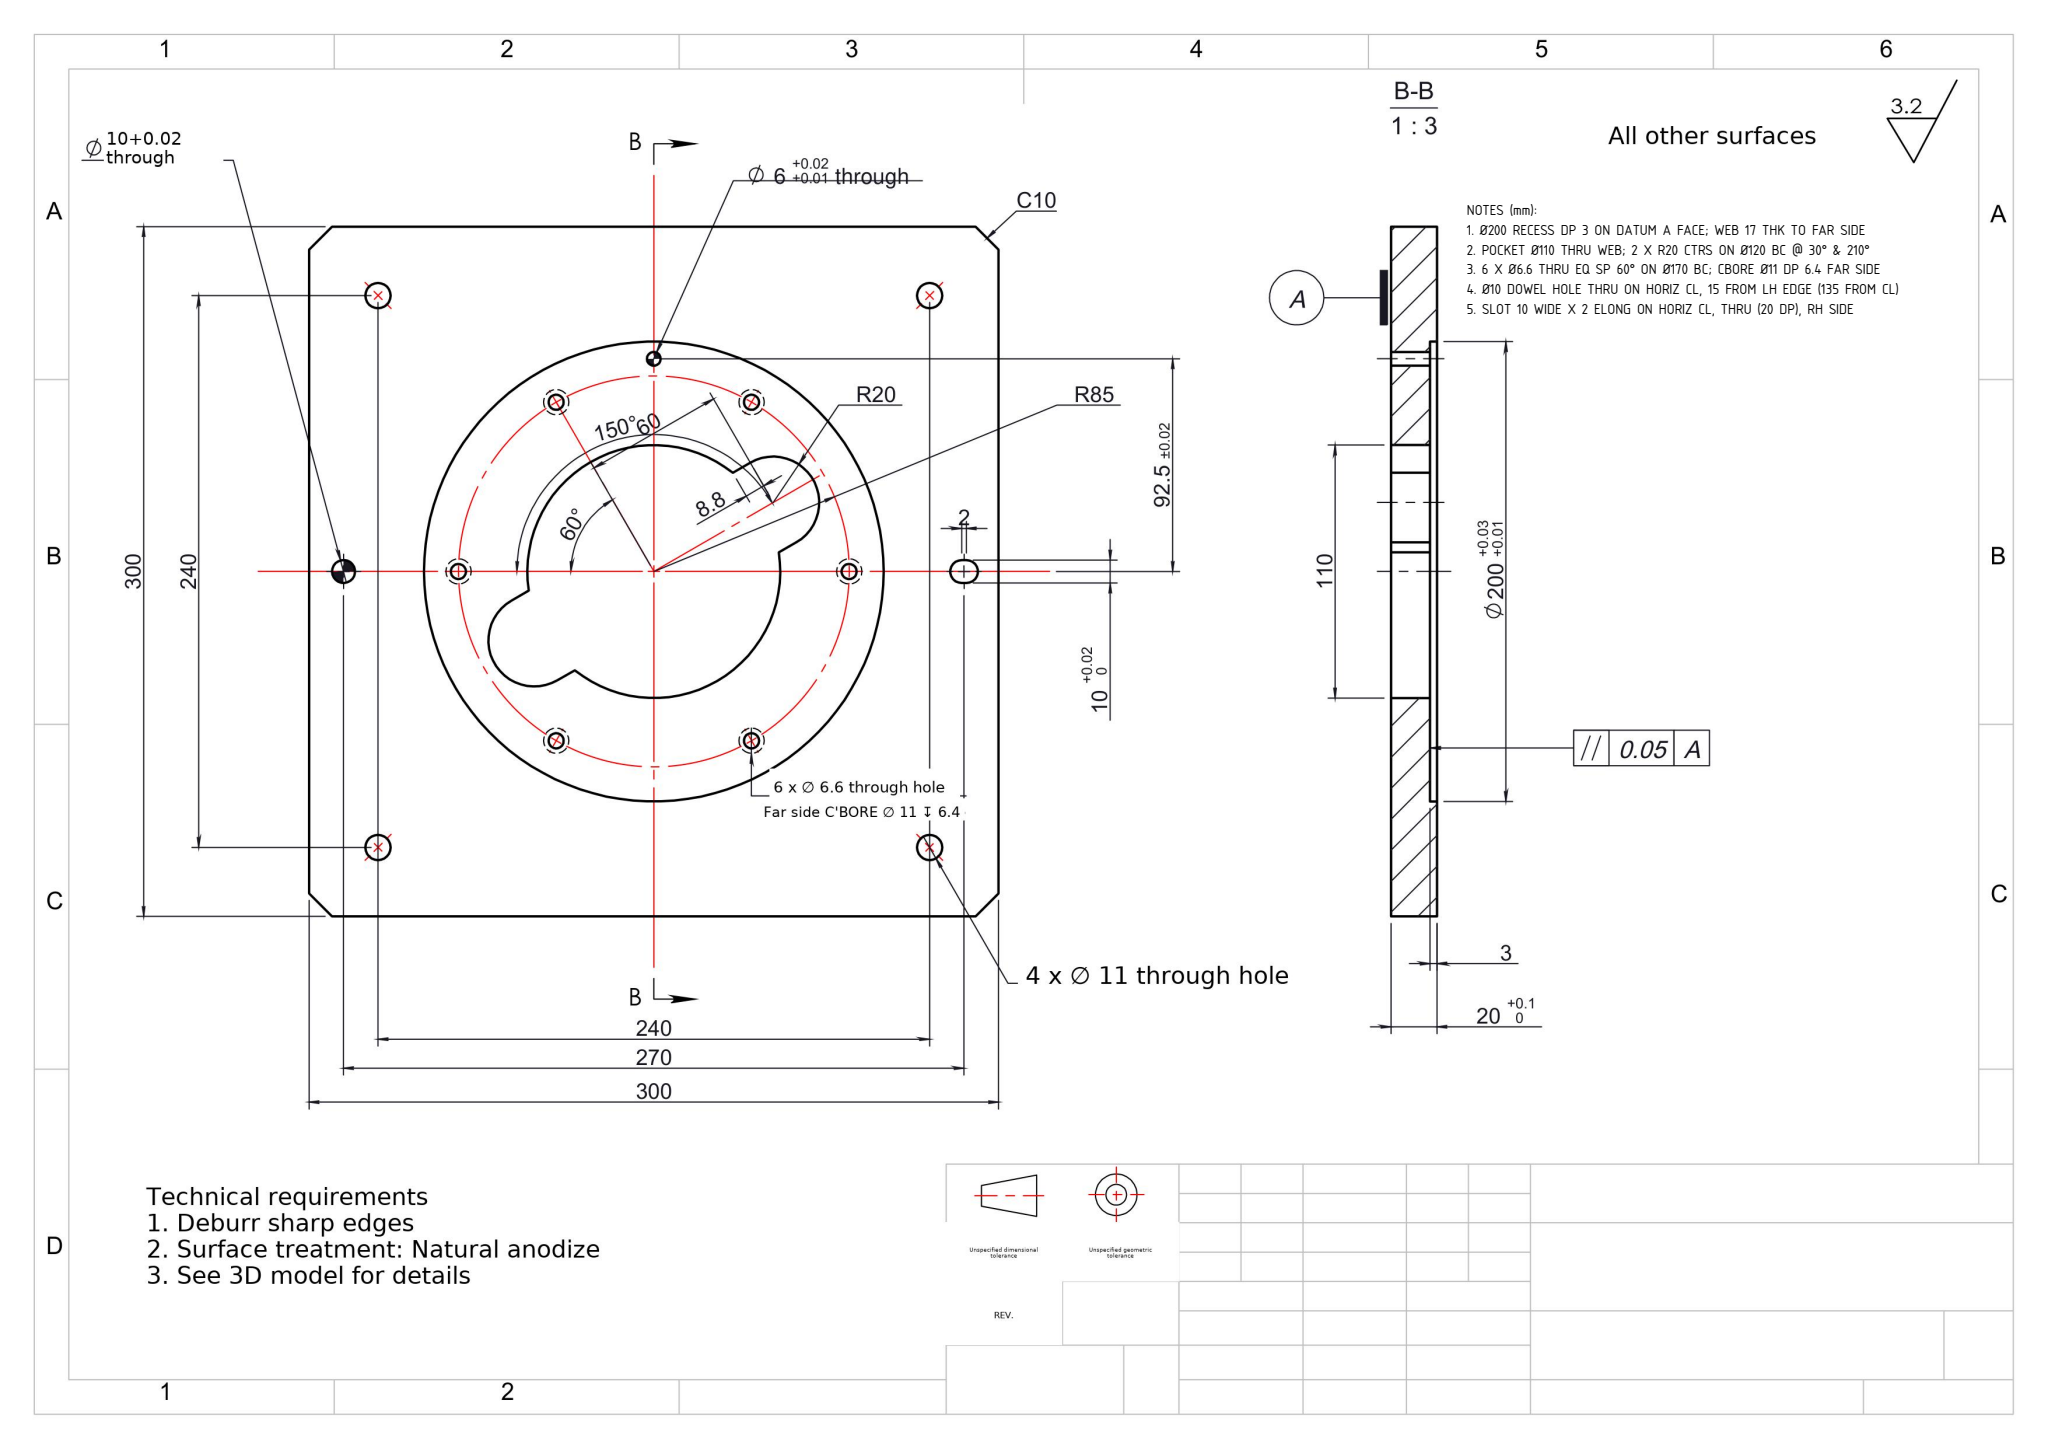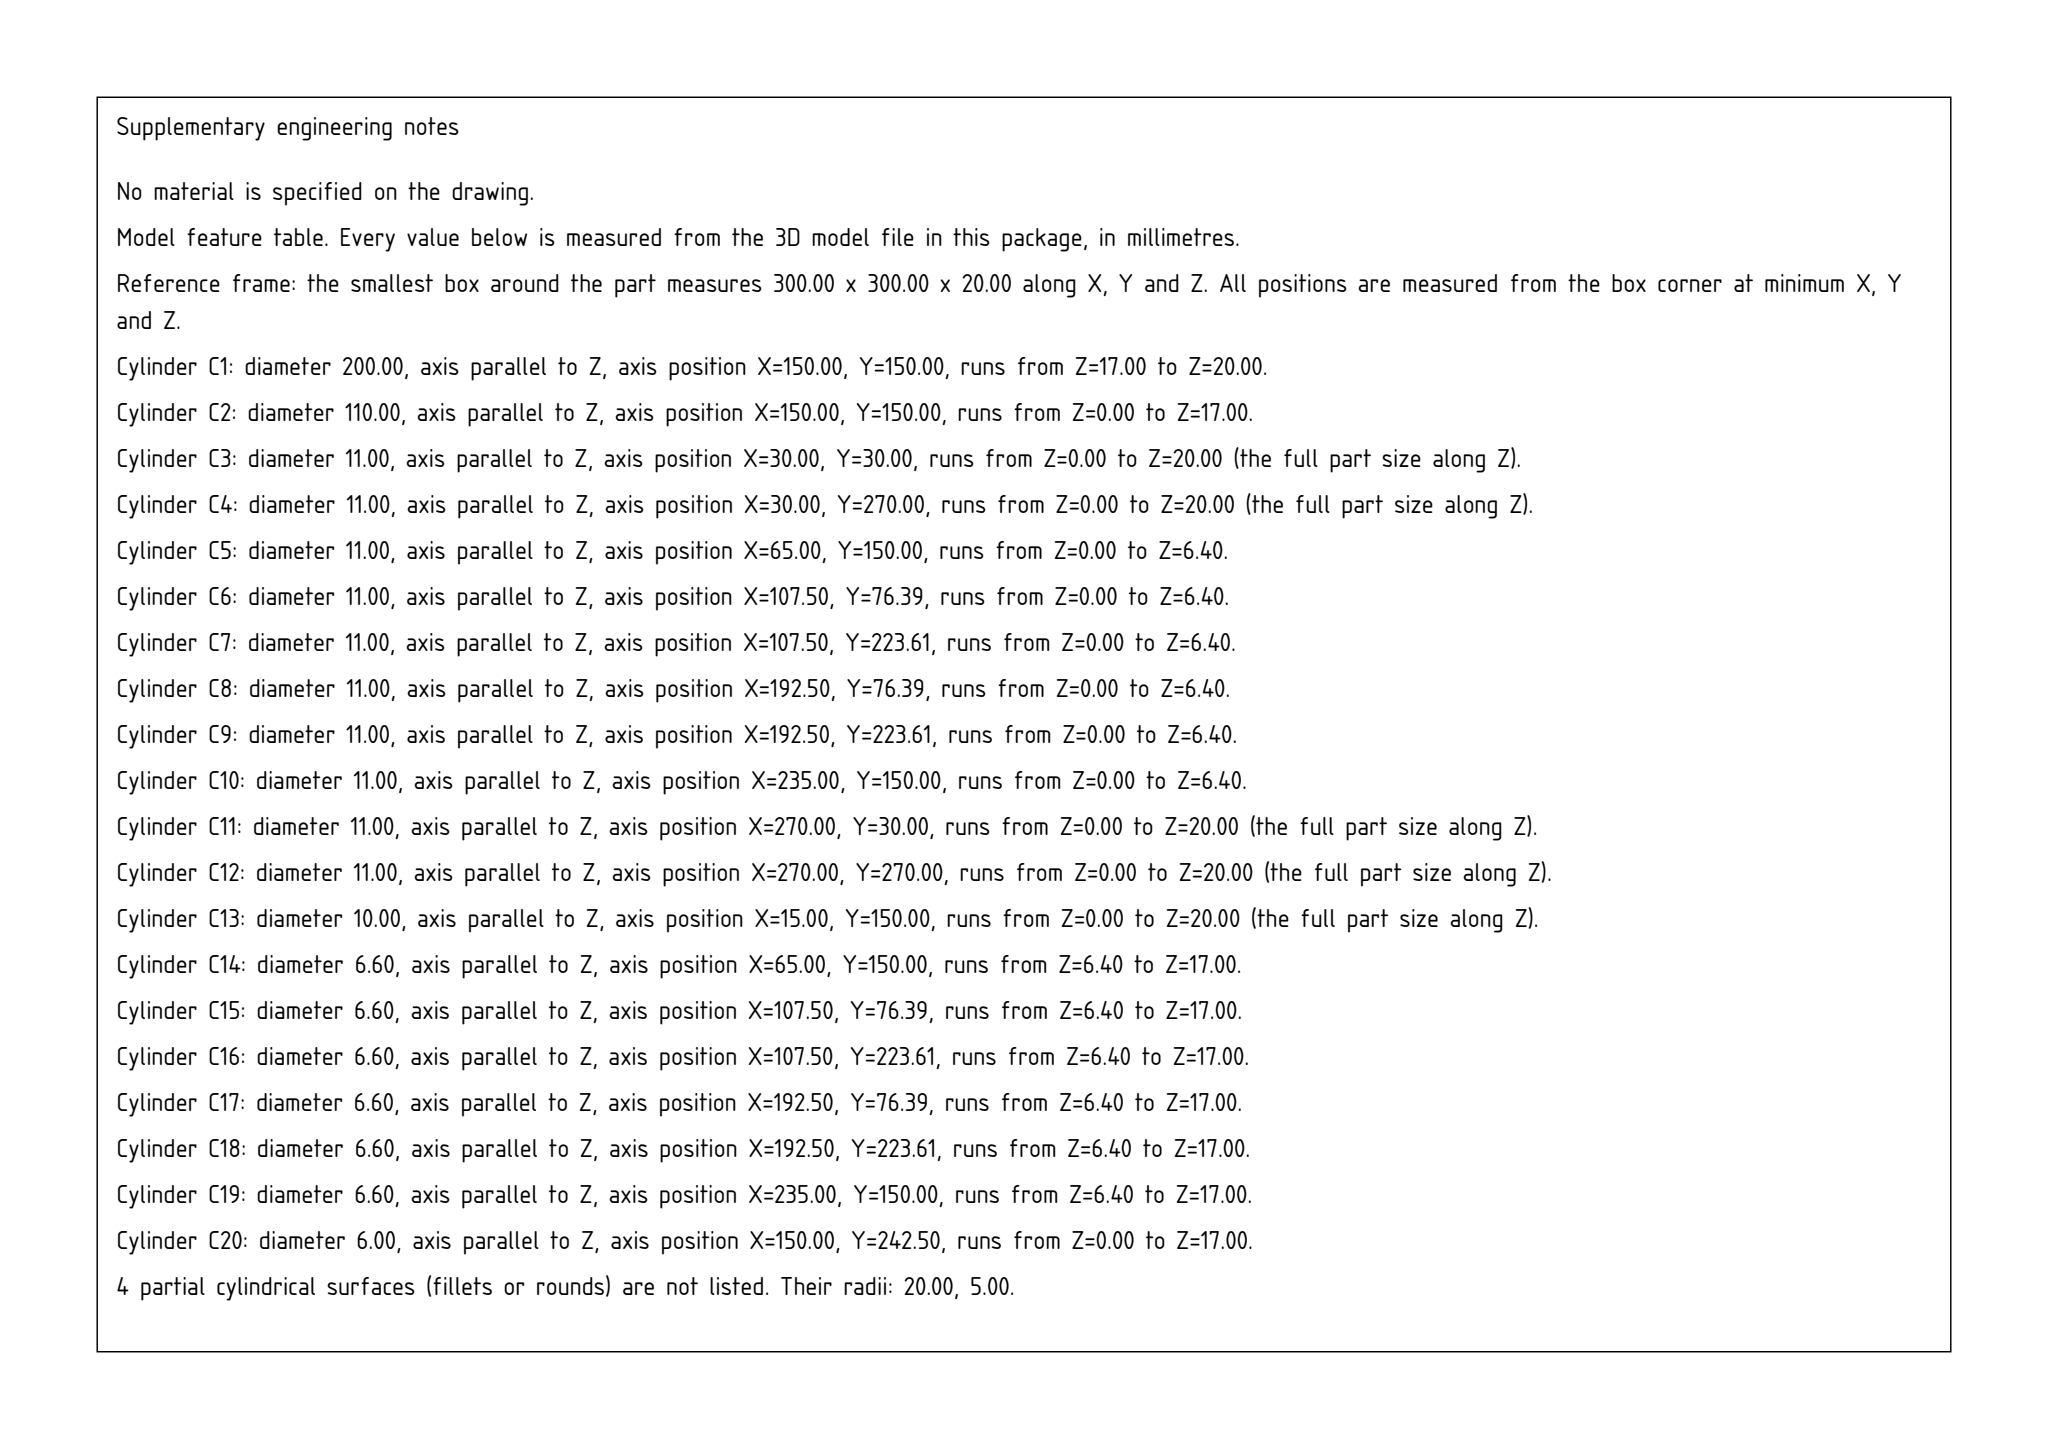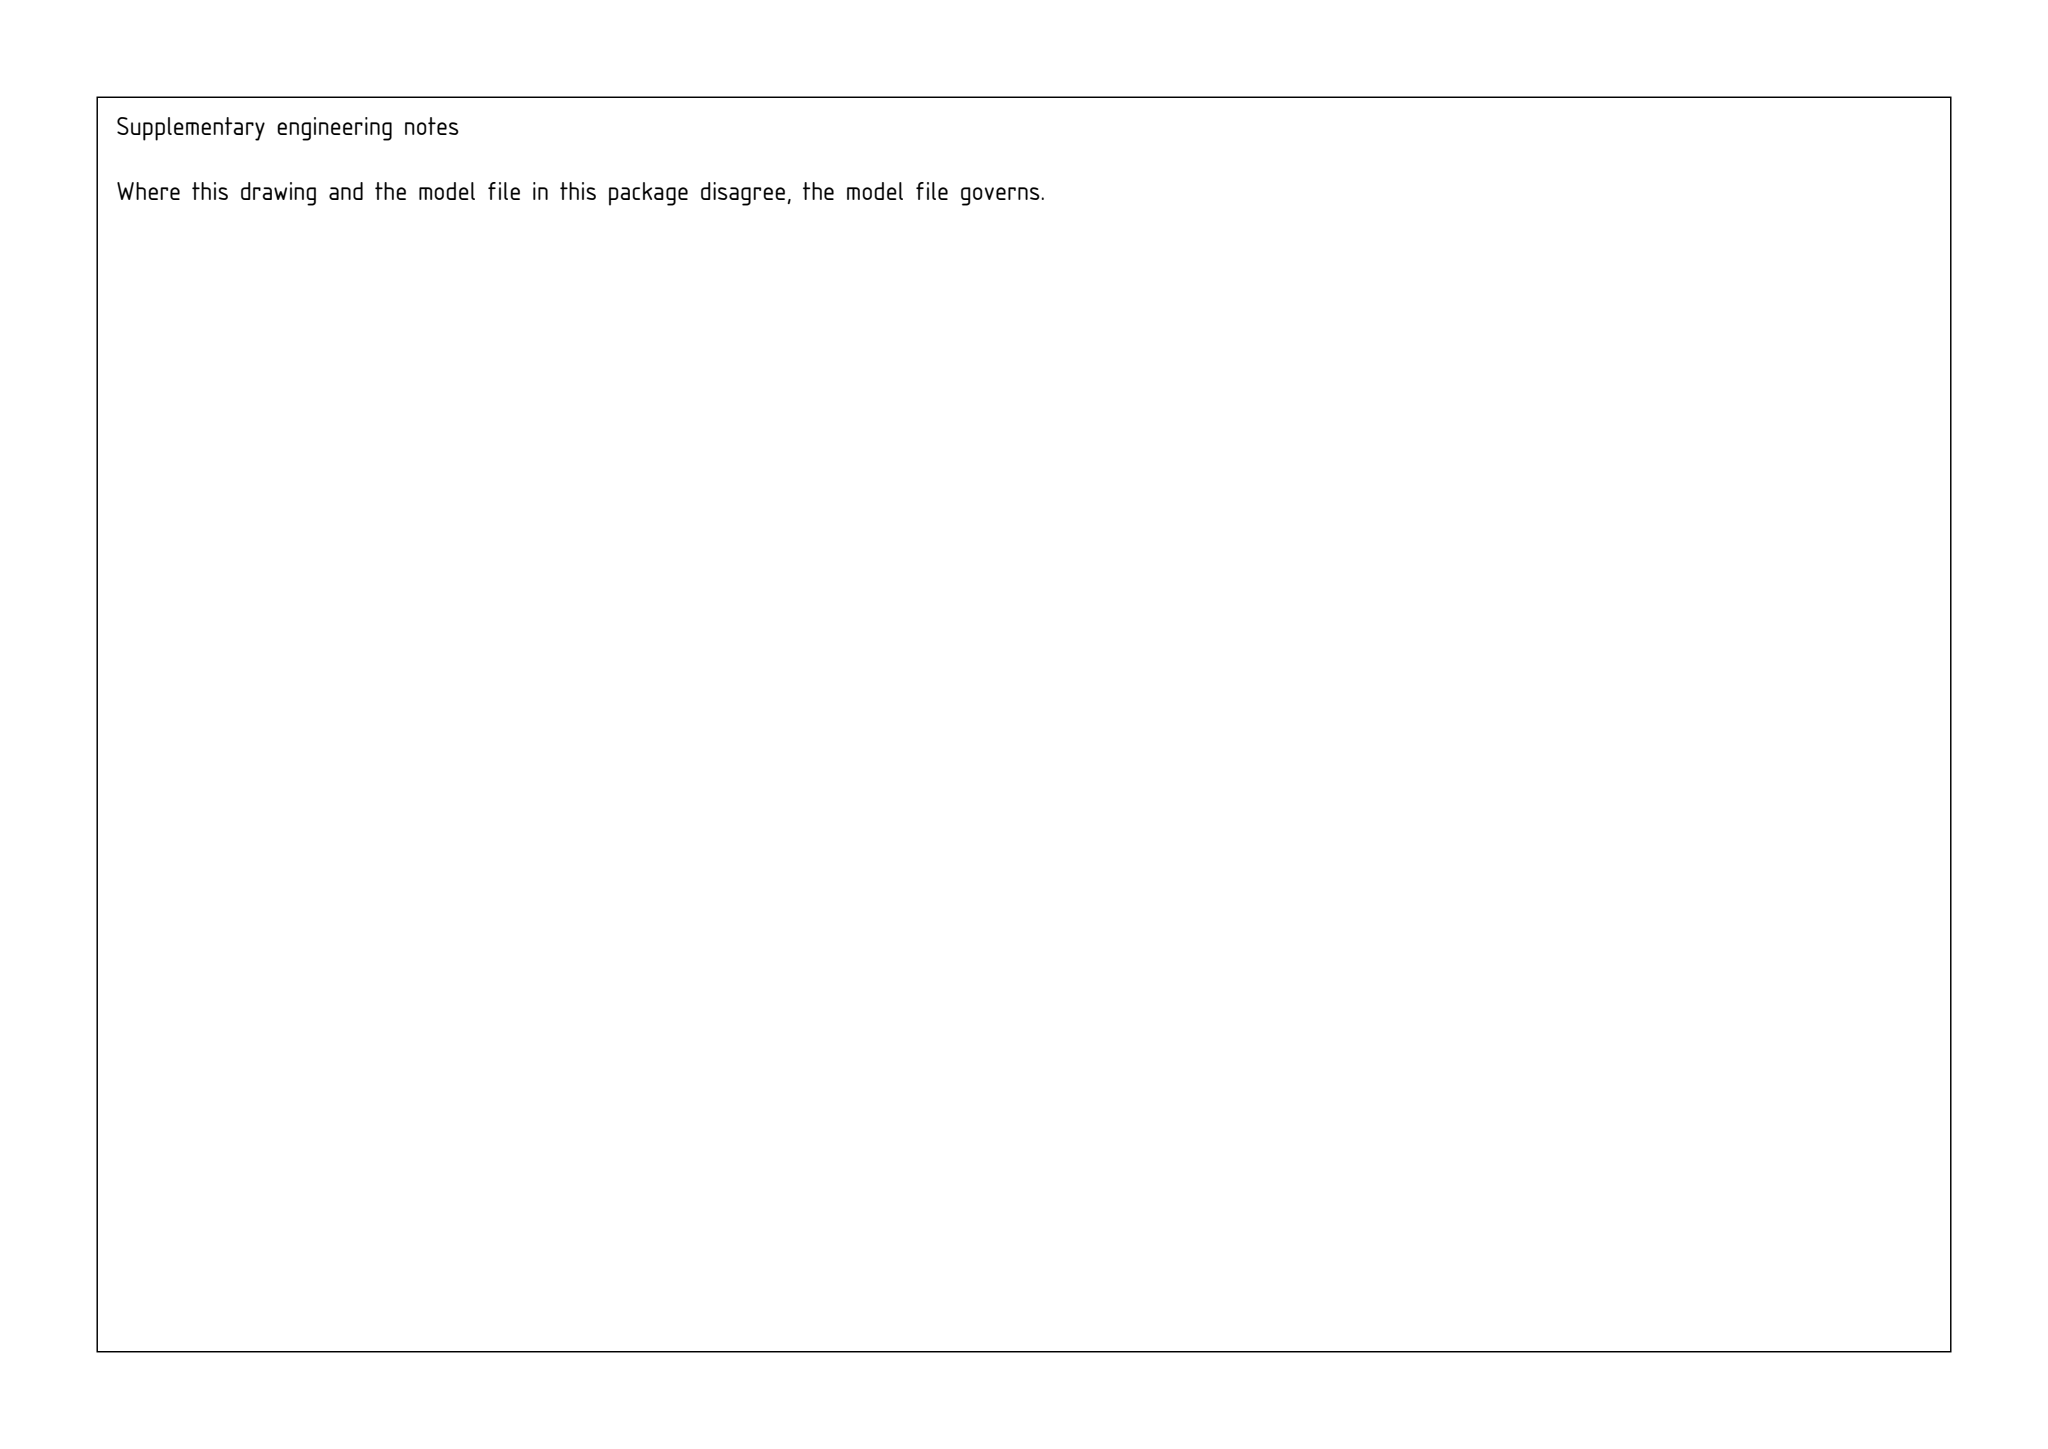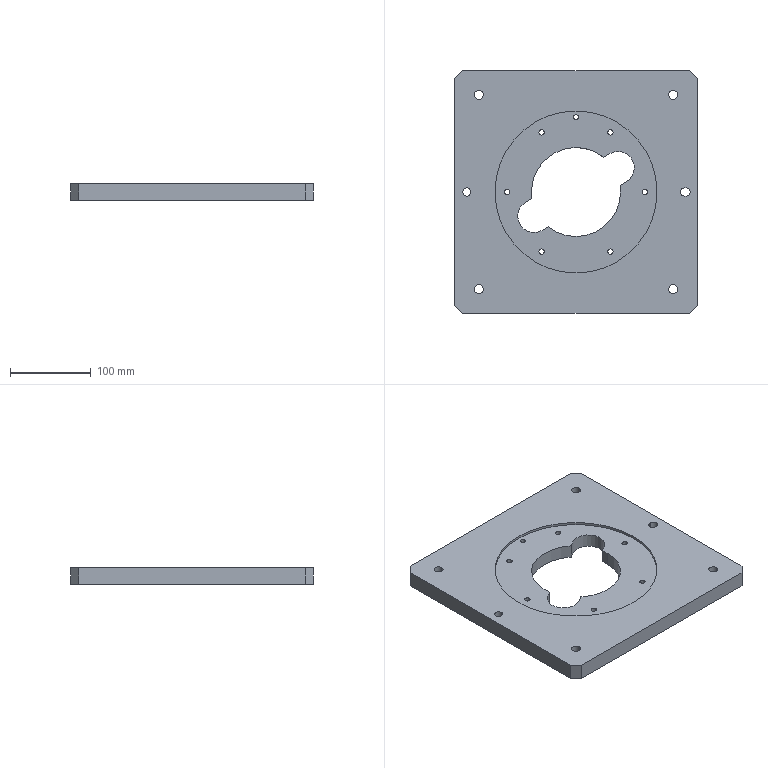Part | SolidWorks | mm | 1 solid | 70 faces | box 300 x 300 x 20 mm | volume 1492900 mm3 | cylinder 47 | plane 23 | commonest cylinder face diameters 11 x20 6.6 x12 10 x5 40 x3 110 x3 6 x2 200 x2
Drawing notes:
Ø200 RECESS DP 3 ON DATUM A FACE; WEB 17 THK TO FAR SIDE | from the solid: Ø200 cyl L3 of 20 thk plate; cut floor plane z=17
POCKET Ø110 THRU WEB; 2 X R20 CTRS ON Ø120 BC @ 30° & 210° | from the solid: Ø110 cyl at (150,150) L17; Ø40 cyls at (98.04,120) & (201.96,180) = R60 from CL
6 X Ø6.6 THRU EQ SP 60° ON Ø170 BC; CBORE Ø11 DP 6.4 FAR SIDE | from the solid: Ø6.6 at (65,150),(235,150),(107.5/192.5, 76.39/223.61) = R85 from (150,150); Ø11 L6.4
Ø10 DOWEL HOLE THRU ON HORIZ CL, 15 FROM LH EDGE (135 FROM CL) | from the solid: Ø10 cyl at (15,150), L20 = full plate thk
SLOT 10 WIDE X 2 ELONG ON HORIZ CL, THRU (20 DP), RH SIDE | from the solid: Ø10 z-cyls at (284,150) & (286,150), L20 = full 20 thk plate
build123d program:
from build123d import *

# Parameters (mm, degrees)
SKETCH1_W                                       = 300
SKETCH1_H                                       = 300
BOSS_EXTRUDE1_DEPTH                             = 20
SKETCH2_R                                       = 100
CUT_EXTRUDE1_DEPTH                              = 3
SKETCH3_R                                       = 55
CUT_EXTRUDE2_DEPTH                              = 213.812
M6_HEX_SOCKET_HEAD_CAP_SCREW_CBORE1_D           = 6.6
M6_HEX_SOCKET_HEAD_CAP_SCREW_CBORE1_CBORE_D     = 11
M6_HEX_SOCKET_HEAD_CAP_SCREW_CBORE1_CBORE_DEPTH = 6.4
CIRPATTERN1_COUNT                               = 6
SIZE_MM_DOWEL_PIN_HOLE1_D                       = 6
CUT_EXTRUDE3_DEPTH                              = 214.073
M10_CLEARANCE_HOLE1_D                           = 11
CIRPATTERN2_COUNT                               = 4
SKETCH11_R                                      = 5
CUT_EXTRUDE4_DEPTH                              = 214.073
CHAMFER1_SIZE                                   = 10


with BuildPart() as part:
    # Sketch1 → Boss-Extrude1 (new body)
    with BuildSketch(Plane.XY):
        Rectangle(SKETCH1_W, SKETCH1_H)
    extrude(amount=BOSS_EXTRUDE1_DEPTH)

    # Sketch2 → Cut-Extrude1 (cut)
    with BuildSketch(Plane.XY.offset(20)):
        Circle(SKETCH2_R)
    extrude(amount=-CUT_EXTRUDE1_DEPTH, mode=Mode.SUBTRACT)

    # Sketch3 → Cut-Extrude2 (cut, through all)
    with BuildSketch(Plane.XY.offset(17)):
        Circle(SKETCH3_R)
    extrude(amount=-CUT_EXTRUDE2_DEPTH, mode=Mode.SUBTRACT)

    # M6 Hex Socket Head Cap Screw CBORE1 (through all)
    with Locations(Plane(origin=(0, 0, 0), x_dir=(-1, 0, 0), z_dir=(0, 0, -1))):
        with Locations((-85, 0)):
            m6_hex_socket_head_cap_screw_cbore1 = CounterBoreHole(M6_HEX_SOCKET_HEAD_CAP_SCREW_CBORE1_D / 2, M6_HEX_SOCKET_HEAD_CAP_SCREW_CBORE1_CBORE_D / 2, M6_HEX_SOCKET_HEAD_CAP_SCREW_CBORE1_CBORE_DEPTH)

    # CirPattern1: M6 Hex Socket Head Cap Screw CBORE1 ×6 about axis
    cirpattern1_axis = Axis((0, 0, 0), (0, 0, 1))
    for i in range(1, CIRPATTERN1_COUNT):
        add(m6_hex_socket_head_cap_screw_cbore1.rotate(cirpattern1_axis, i * 360 / CIRPATTERN1_COUNT), mode=Mode.SUBTRACT)

    # Size mm Dowel Pin Hole1 (through all)
    with Locations(Plane(origin=(0, 0, 0), x_dir=(-1, 0, 0), z_dir=(0, 0, -1))):
        with Locations((0, 92.5)):
            Hole(SIZE_MM_DOWEL_PIN_HOLE1_D / 2)

    # Sketch8 → Cut-Extrude3 (cut, through all)
    with BuildSketch(Plane(origin=(0, 0, 0), x_dir=(-1, 0, 0), z_dir=(0, 0, -1))):
        with BuildLine():
            Line((-41.962, 47.321), (61.962, -12.679))
            ThreePointArc((61.962, -12.679), (69.282, -40), (41.962, -47.321))
            Line((41.962, -47.321), (-61.962, 12.679))
            ThreePointArc((-61.962, 12.679), (-69.282, 40), (-41.962, 47.321))
        make_face()
    extrude(amount=-CUT_EXTRUDE3_DEPTH, mode=Mode.SUBTRACT)

    # M10 Clearance Hole1 (through all)
    with Locations(Plane(origin=(0, 0, 0), x_dir=(-1, 0, 0), z_dir=(0, 0, -1))):
        with Locations((-120, 120)):
            m10_clearance_hole1 = Hole(M10_CLEARANCE_HOLE1_D / 2)

    # CirPattern2: M10 Clearance Hole1 ×4 about axis
    cirpattern2_axis = Axis((0, 0, 0), (0, 0, 1))
    for i in range(1, CIRPATTERN2_COUNT):
        add(m10_clearance_hole1.rotate(cirpattern2_axis, i * 360 / CIRPATTERN2_COUNT), mode=Mode.SUBTRACT)

    # Sketch11 → Cut-Extrude4 (cut, through all)
    with BuildSketch(Plane(origin=(0, 0, 0), x_dir=(-1, 0, 0), z_dir=(0, 0, -1))):
        with Locations((135, 0)):
            Circle(SKETCH11_R)
        with BuildLine():
            Line((-134, -5), (-136, -5))
            ThreePointArc((-136, -5), (-141, 0), (-136, 5))
            Line((-136, 5), (-134, 5))
            ThreePointArc((-134, 5), (-129, 0), (-134, -5))
        make_face()
    extrude(amount=-CUT_EXTRUDE4_DEPTH, mode=Mode.SUBTRACT)

    # Chamfer1
    chamfer1_edges = [part.edges().sort_by_distance(p)[0] for p in [
        (150, -150, 10),
        (-150, -150, 10),
        (-150, 150, 10),
        (150, 150, 10),
    ]]
    chamfer(chamfer1_edges, length=CHAMFER1_SIZE)


solid = part.part